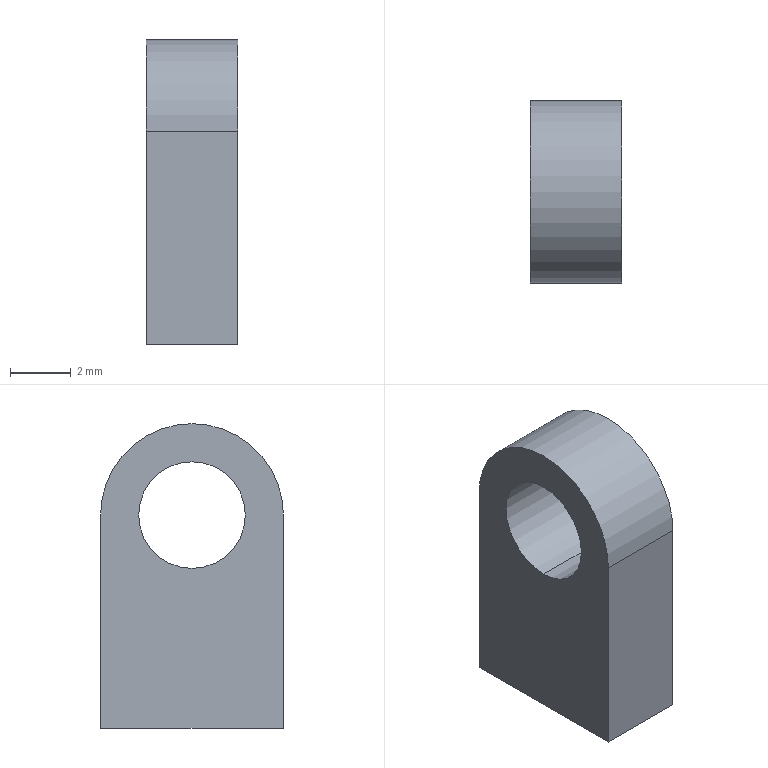Component | SolidWorks | MGL-PACK-03-00Fixture-1_MGL-PACK-03-03SpringSeat-1 | 1 solid | 8 faces | box 3 x 6 x 10 mm | volume 140 mm3 | plane 5 | cylinder 3 | commonest cylinder face diameters 3.5 x2 6 x1
build123d program:
from build123d import *

# Parameters (mm, degrees)
SKETCH1_R           = 1.75
BOSS_EXTRUDE1_DEPTH = 3


with BuildPart() as part:
    # Sketch1 → Boss-Extrude1 (new body)
    with BuildSketch(Plane.XY):
        with BuildLine():
            Line((-3.5, 3), (3.5, 3))
            ThreePointArc((3.5, 3), (6.5, 0), (3.5, -3))
            Line((3.5, -3), (-3.5, -3))
            Line((-3.5, -3), (-3.5, 3))
        make_face()
        with Locations((3.5, 0)):
            Circle(SKETCH1_R, mode=Mode.SUBTRACT)
    extrude(amount=BOSS_EXTRUDE1_DEPTH)


solid = part.part

# Placed as in the assembly
solid = solid.moved(Location((235.5, 72, -261.8), (0, -90, 0)))
STEP:
#1=COLOUR_RGB('',0.7922,0.8196,0.9333);
#2=FILL_AREA_STYLE_COLOUR('',#1);
#3=FILL_AREA_STYLE('',(#2));
#4=SURFACE_STYLE_FILL_AREA(#3);
#5=SURFACE_SIDE_STYLE('',(#4));
#6=SURFACE_STYLE_USAGE(.BOTH.,#5);
#7=PRESENTATION_STYLE_ASSIGNMENT((#6));
#8=CARTESIAN_POINT('',(9.154,2.835,-10.238));
#9=VERTEX_POINT('',#8);
#10=CARTESIAN_POINT('',(9.154,2.835,-10.1));
#11=VERTEX_POINT('',#10);
#12=CARTESIAN_POINT('',(9.154,2.835,-10.169));
#13=DIRECTION('',(-1.,-0.,0.));
#14=DIRECTION('',(0.,0.,1.));
#15=AXIS2_PLACEMENT_3D('',#12,#13,#14);
#16=CIRCLE('',#15,0.0689);
#17=EDGE_CURVE('',#9,#11,#16,.T.);
#18=ORIENTED_EDGE('',*,*,#17,.T.);
#19=CARTESIAN_POINT('',(9.272,2.835,-10.1));
#20=VERTEX_POINT('',#19);
#21=CARTESIAN_POINT('',(9.154,2.835,-10.1));
#22=DIRECTION('',(1.,0.,-0.));
#23=VECTOR('',#22,39.37);
#24=LINE('',#21,#23);
#25=EDGE_CURVE('',#11,#20,#24,.T.);
#26=ORIENTED_EDGE('',*,*,#25,.T.);
#27=CARTESIAN_POINT('',(9.272,2.835,-10.238));
#28=VERTEX_POINT('',#27);
#29=CARTESIAN_POINT('',(9.272,2.835,-10.169));
#30=DIRECTION('',(-1.,-0.,0.));
#31=DIRECTION('',(0.,0.,1.));
#32=AXIS2_PLACEMENT_3D('',#29,#30,#31);
#33=CIRCLE('',#32,0.0689);
#34=EDGE_CURVE('',#28,#20,#33,.T.);
#35=ORIENTED_EDGE('',*,*,#34,.F.);
#36=CARTESIAN_POINT('',(9.154,2.835,-10.238));
#37=DIRECTION('',(1.,0.,-0.));
#38=VECTOR('',#37,39.37);
#39=LINE('',#36,#38);
#40=EDGE_CURVE('',#9,#28,#39,.T.);
#41=ORIENTED_EDGE('',*,*,#40,.F.);
#42=EDGE_LOOP('',(#18,#26,#35,#41));
#43=FACE_OUTER_BOUND('',#42,.T.);
#44=CARTESIAN_POINT('',(9.154,2.835,-10.169));
#45=DIRECTION('',(1.,0.,-0.));
#46=DIRECTION('',(0.,0.,-1.));
#47=AXIS2_PLACEMENT_3D('',#44,#45,#46);
#48=CYLINDRICAL_SURFACE('',#47,0.0689);
#49=ADVANCED_FACE('',(#43),#48,.F.);
#50=CARTESIAN_POINT('',(9.154,2.953,-10.445));
#51=VERTEX_POINT('',#50);
#52=CARTESIAN_POINT('',(9.154,2.717,-10.445));
#53=VERTEX_POINT('',#52);
#54=CARTESIAN_POINT('',(9.154,2.953,-10.445));
#55=DIRECTION('',(0.,-1.,0.));
#56=VECTOR('',#55,39.37);
#57=LINE('',#54,#56);
#58=EDGE_CURVE('',#51,#53,#57,.T.);
#59=ORIENTED_EDGE('',*,*,#58,.T.);
#60=CARTESIAN_POINT('',(9.154,2.717,-10.169));
#61=VERTEX_POINT('',#60);
#62=CARTESIAN_POINT('',(9.154,2.717,-10.445));
#63=DIRECTION('',(0.,-0.,1.));
#64=VECTOR('',#63,39.37);
#65=LINE('',#62,#64);
#66=EDGE_CURVE('',#53,#61,#65,.T.);
#67=ORIENTED_EDGE('',*,*,#66,.T.);
#68=CARTESIAN_POINT('',(9.154,2.953,-10.169));
#69=VERTEX_POINT('',#68);
#70=CARTESIAN_POINT('',(9.154,2.835,-10.169));
#71=DIRECTION('',(-1.,-0.,0.));
#72=DIRECTION('',(0.,0.,1.));
#73=AXIS2_PLACEMENT_3D('',#70,#71,#72);
#74=CIRCLE('',#73,0.1181);
#75=EDGE_CURVE('',#61,#69,#74,.T.);
#76=ORIENTED_EDGE('',*,*,#75,.T.);
#77=CARTESIAN_POINT('',(9.154,2.953,-10.445));
#78=DIRECTION('',(-0.,-0.,-1.));
#79=VECTOR('',#78,39.37);
#80=LINE('',#77,#79);
#81=EDGE_CURVE('',#69,#51,#80,.T.);
#82=ORIENTED_EDGE('',*,*,#81,.T.);
#83=EDGE_LOOP('',(#59,#67,#76,#82));
#84=FACE_OUTER_BOUND('',#83,.T.);
#85=ORIENTED_EDGE('',*,*,#17,.F.);
#86=CARTESIAN_POINT('',(9.154,2.835,-10.169));
#87=DIRECTION('',(-1.,-0.,0.));
#88=DIRECTION('',(0.,0.,1.));
#89=AXIS2_PLACEMENT_3D('',#86,#87,#88);
#90=CIRCLE('',#89,0.0689);
#91=EDGE_CURVE('',#11,#9,#90,.T.);
#92=ORIENTED_EDGE('',*,*,#91,.F.);
#93=EDGE_LOOP('',(#85,#92));
#94=FACE_BOUND('',#93,.T.);
#95=CARTESIAN_POINT('',(9.154,2.835,-10.169));
#96=DIRECTION('',(-1.,-0.,0.));
#97=DIRECTION('',(0.,-0.,1.));
#98=AXIS2_PLACEMENT_3D('',#95,#96,#97);
#99=PLANE('',#98);
#100=ADVANCED_FACE('',(#84,#94),#99,.T.);
#101=CARTESIAN_POINT('',(9.272,2.953,-10.445));
#102=VERTEX_POINT('',#101);
#103=CARTESIAN_POINT('',(9.272,2.717,-10.445));
#104=VERTEX_POINT('',#103);
#105=CARTESIAN_POINT('',(9.272,2.953,-10.445));
#106=DIRECTION('',(0.,-1.,0.));
#107=VECTOR('',#106,39.37);
#108=LINE('',#105,#107);
#109=EDGE_CURVE('',#102,#104,#108,.T.);
#110=ORIENTED_EDGE('',*,*,#109,.F.);
#111=CARTESIAN_POINT('',(9.272,2.953,-10.169));
#112=VERTEX_POINT('',#111);
#113=CARTESIAN_POINT('',(9.272,2.953,-10.445));
#114=DIRECTION('',(-0.,-0.,-1.));
#115=VECTOR('',#114,39.37);
#116=LINE('',#113,#115);
#117=EDGE_CURVE('',#112,#102,#116,.T.);
#118=ORIENTED_EDGE('',*,*,#117,.F.);
#119=CARTESIAN_POINT('',(9.272,2.717,-10.169));
#120=VERTEX_POINT('',#119);
#121=CARTESIAN_POINT('',(9.272,2.835,-10.169));
#122=DIRECTION('',(-1.,-0.,0.));
#123=DIRECTION('',(0.,0.,1.));
#124=AXIS2_PLACEMENT_3D('',#121,#122,#123);
#125=CIRCLE('',#124,0.1181);
#126=EDGE_CURVE('',#120,#112,#125,.T.);
#127=ORIENTED_EDGE('',*,*,#126,.F.);
#128=CARTESIAN_POINT('',(9.272,2.717,-10.445));
#129=DIRECTION('',(0.,-0.,1.));
#130=VECTOR('',#129,39.37);
#131=LINE('',#128,#130);
#132=EDGE_CURVE('',#104,#120,#131,.T.);
#133=ORIENTED_EDGE('',*,*,#132,.F.);
#134=EDGE_LOOP('',(#110,#118,#127,#133));
#135=FACE_OUTER_BOUND('',#134,.T.);
#136=ORIENTED_EDGE('',*,*,#34,.T.);
#137=CARTESIAN_POINT('',(9.272,2.835,-10.169));
#138=DIRECTION('',(-1.,-0.,0.));
#139=DIRECTION('',(0.,0.,1.));
#140=AXIS2_PLACEMENT_3D('',#137,#138,#139);
#141=CIRCLE('',#140,0.0689);
#142=EDGE_CURVE('',#20,#28,#141,.T.);
#143=ORIENTED_EDGE('',*,*,#142,.T.);
#144=EDGE_LOOP('',(#136,#143));
#145=FACE_BOUND('',#144,.T.);
#146=CARTESIAN_POINT('',(9.272,2.835,-10.169));
#147=DIRECTION('',(-1.,-0.,0.));
#148=DIRECTION('',(0.,-0.,1.));
#149=AXIS2_PLACEMENT_3D('',#146,#147,#148);
#150=PLANE('',#149);
#151=ADVANCED_FACE('',(#135,#145),#150,.F.);
#152=ORIENTED_EDGE('',*,*,#109,.T.);
#153=CARTESIAN_POINT('',(9.154,2.717,-10.445));
#154=DIRECTION('',(1.,0.,-0.));
#155=VECTOR('',#154,39.37);
#156=LINE('',#153,#155);
#157=EDGE_CURVE('',#53,#104,#156,.T.);
#158=ORIENTED_EDGE('',*,*,#157,.F.);
#159=ORIENTED_EDGE('',*,*,#58,.F.);
#160=CARTESIAN_POINT('',(9.154,2.953,-10.445));
#161=DIRECTION('',(1.,0.,-0.));
#162=VECTOR('',#161,39.37);
#163=LINE('',#160,#162);
#164=EDGE_CURVE('',#51,#102,#163,.T.);
#165=ORIENTED_EDGE('',*,*,#164,.T.);
#166=EDGE_LOOP('',(#152,#158,#159,#165));
#167=FACE_OUTER_BOUND('',#166,.T.);
#168=CARTESIAN_POINT('',(9.154,2.953,-10.445));
#169=DIRECTION('',(0.,0.,1.));
#170=DIRECTION('',(-0.,1.,-0.));
#171=AXIS2_PLACEMENT_3D('',#168,#169,#170);
#172=PLANE('',#171);
#173=ADVANCED_FACE('',(#167),#172,.F.);
#174=ORIENTED_EDGE('',*,*,#132,.T.);
#175=CARTESIAN_POINT('',(9.154,2.717,-10.169));
#176=DIRECTION('',(1.,0.,-0.));
#177=VECTOR('',#176,39.37);
#178=LINE('',#175,#177);
#179=EDGE_CURVE('',#61,#120,#178,.T.);
#180=ORIENTED_EDGE('',*,*,#179,.F.);
#181=ORIENTED_EDGE('',*,*,#66,.F.);
#182=ORIENTED_EDGE('',*,*,#157,.T.);
#183=EDGE_LOOP('',(#174,#180,#181,#182));
#184=FACE_OUTER_BOUND('',#183,.T.);
#185=CARTESIAN_POINT('',(9.154,2.717,-10.445));
#186=DIRECTION('',(-0.,1.,0.));
#187=DIRECTION('',(-1.,-0.,0.));
#188=AXIS2_PLACEMENT_3D('',#185,#186,#187);
#189=PLANE('',#188);
#190=ADVANCED_FACE('',(#184),#189,.F.);
#191=ORIENTED_EDGE('',*,*,#126,.T.);
#192=CARTESIAN_POINT('',(9.154,2.953,-10.169));
#193=DIRECTION('',(1.,0.,-0.));
#194=VECTOR('',#193,39.37);
#195=LINE('',#192,#194);
#196=EDGE_CURVE('',#69,#112,#195,.T.);
#197=ORIENTED_EDGE('',*,*,#196,.F.);
#198=ORIENTED_EDGE('',*,*,#75,.F.);
#199=ORIENTED_EDGE('',*,*,#179,.T.);
#200=EDGE_LOOP('',(#191,#197,#198,#199));
#201=FACE_OUTER_BOUND('',#200,.T.);
#202=CARTESIAN_POINT('',(9.154,2.835,-10.169));
#203=DIRECTION('',(1.,0.,-0.));
#204=DIRECTION('',(0.,0.,-1.));
#205=AXIS2_PLACEMENT_3D('',#202,#203,#204);
#206=CYLINDRICAL_SURFACE('',#205,0.1181);
#207=ADVANCED_FACE('',(#201),#206,.T.);
#208=ORIENTED_EDGE('',*,*,#117,.T.);
#209=ORIENTED_EDGE('',*,*,#164,.F.);
#210=ORIENTED_EDGE('',*,*,#81,.F.);
#211=ORIENTED_EDGE('',*,*,#196,.T.);
#212=EDGE_LOOP('',(#208,#209,#210,#211));
#213=FACE_OUTER_BOUND('',#212,.T.);
#214=CARTESIAN_POINT('',(9.154,2.953,-10.445));
#215=DIRECTION('',(0.,-1.,0.));
#216=DIRECTION('',(0.,0.,1.));
#217=AXIS2_PLACEMENT_3D('',#214,#215,#216);
#218=PLANE('',#217);
#219=ADVANCED_FACE('',(#213),#218,.F.);
#220=ORIENTED_EDGE('',*,*,#25,.F.);
#221=ORIENTED_EDGE('',*,*,#91,.T.);
#222=ORIENTED_EDGE('',*,*,#40,.T.);
#223=ORIENTED_EDGE('',*,*,#142,.F.);
#224=EDGE_LOOP('',(#220,#221,#222,#223));
#225=FACE_OUTER_BOUND('',#224,.T.);
#226=CARTESIAN_POINT('',(9.154,2.835,-10.169));
#227=DIRECTION('',(1.,0.,-0.));
#228=DIRECTION('',(0.,0.,-1.));
#229=AXIS2_PLACEMENT_3D('',#226,#227,#228);
#230=CYLINDRICAL_SURFACE('',#229,0.0689);
#231=ADVANCED_FACE('',(#225),#230,.F.);
#232=CLOSED_SHELL('',(#49,#100,#151,#173,#190,#207,#219,#231));
#233=MANIFOLD_SOLID_BREP('',#232);
#234=STYLED_ITEM('',(#7),#233);
#235=PRESENTATION_LAYER_ASSIGNMENT('','',(#234));
#236=(LENGTH_UNIT()NAMED_UNIT(*)SI_UNIT($,.METRE.));
#237=LENGTH_MEASURE_WITH_UNIT(LENGTH_MEASURE(0.0254),#236);
#238=DIMENSIONAL_EXPONENTS(1.,0.,0.,0.,0.,0.,0.);
#239=(CONVERSION_BASED_UNIT('',#237)LENGTH_UNIT()NAMED_UNIT(#238));
#240=UNCERTAINTY_MEASURE_WITH_UNIT(LENGTH_MEASURE(0.00001),#239,'','');
#241=(NAMED_UNIT(*)PLANE_ANGLE_UNIT()SI_UNIT($,.RADIAN.));
#242=(NAMED_UNIT(*)SI_UNIT($,.STERADIAN.)SOLID_ANGLE_UNIT());
#243=(GEOMETRIC_REPRESENTATION_CONTEXT(3)GLOBAL_UNCERTAINTY_ASSIGNED_CONTEXT((#240))GLOBAL_UNIT_ASSIGNED_CONTEXT((#239,#241,#242))REPRESENTATION_CONTEXT('',''));
#244=MECHANICAL_DESIGN_GEOMETRIC_PRESENTATION_REPRESENTATION('',(#234),#243);
#245=CARTESIAN_POINT('',(0.,0.,0.));
#246=DIRECTION('',(0.,0.,1.));
#247=DIRECTION('',(1.,0.,0.));
#248=AXIS2_PLACEMENT_3D('',#245,#246,#247);
#249=(LENGTH_UNIT()NAMED_UNIT(*)SI_UNIT($,.METRE.));
#250=LENGTH_MEASURE_WITH_UNIT(LENGTH_MEASURE(0.0254),#249);
#251=DIMENSIONAL_EXPONENTS(1.,0.,0.,0.,0.,0.,0.);
#252=(CONVERSION_BASED_UNIT('',#250)LENGTH_UNIT()NAMED_UNIT(#251));
#253=UNCERTAINTY_MEASURE_WITH_UNIT(LENGTH_MEASURE(0.00001),#252,'','');
#254=(NAMED_UNIT(*)PLANE_ANGLE_UNIT()SI_UNIT($,.RADIAN.));
#255=(NAMED_UNIT(*)SI_UNIT($,.STERADIAN.)SOLID_ANGLE_UNIT());
#256=(GEOMETRIC_REPRESENTATION_CONTEXT(3)GLOBAL_UNCERTAINTY_ASSIGNED_CONTEXT((#253))GLOBAL_UNIT_ASSIGNED_CONTEXT((#252,#254,#255))REPRESENTATION_CONTEXT('',''));
#257=ADVANCED_BREP_SHAPE_REPRESENTATION('',(#233,#248),#256);